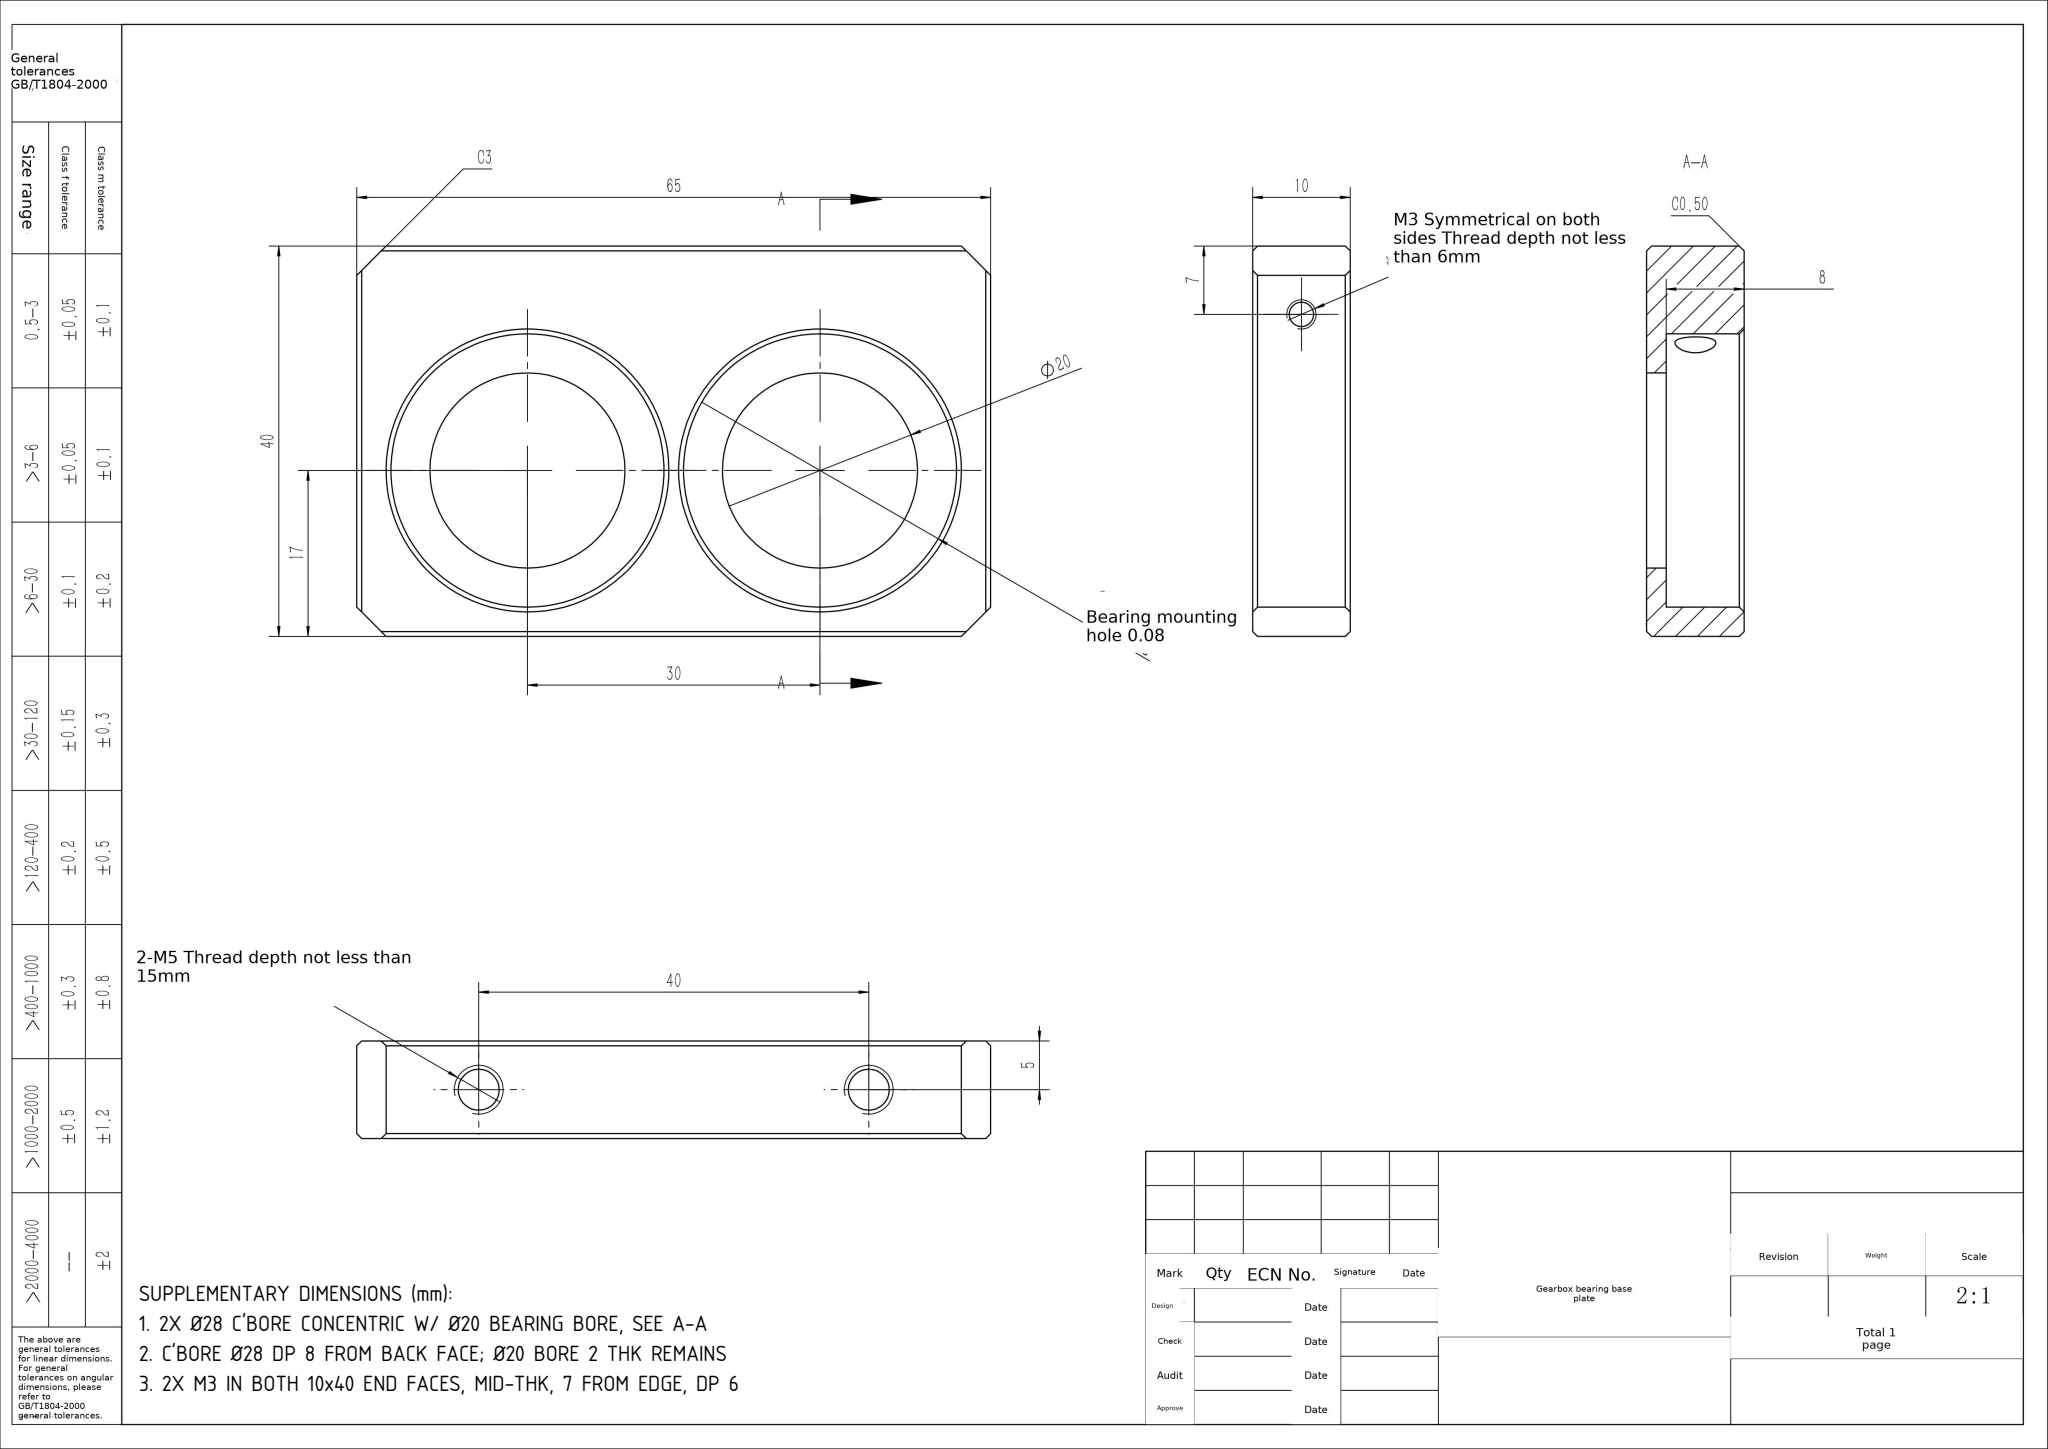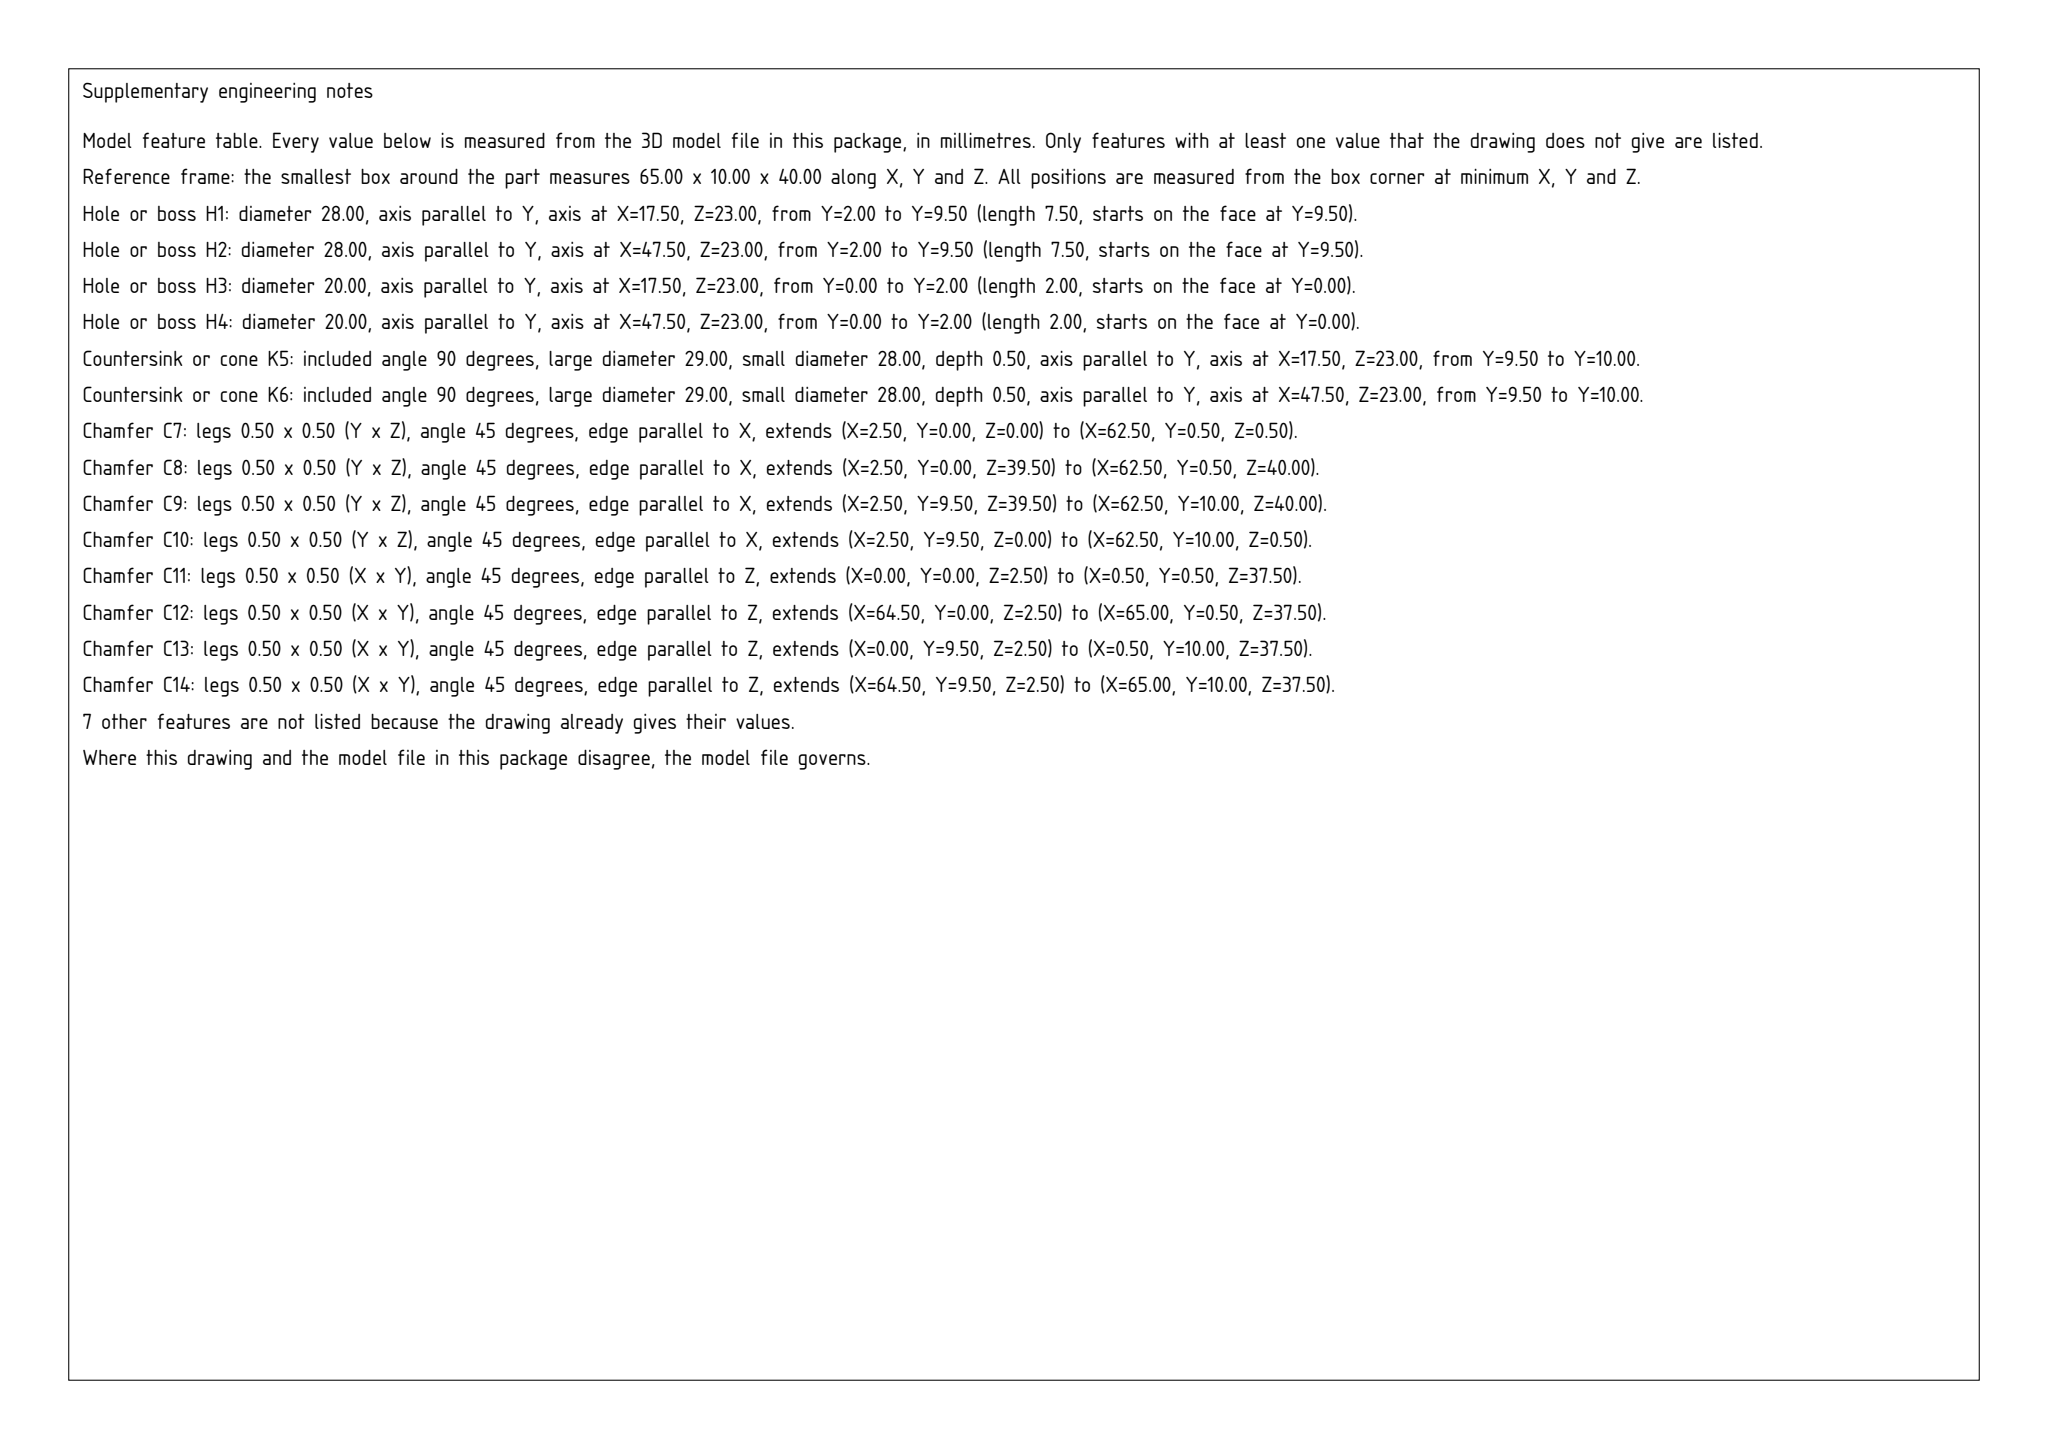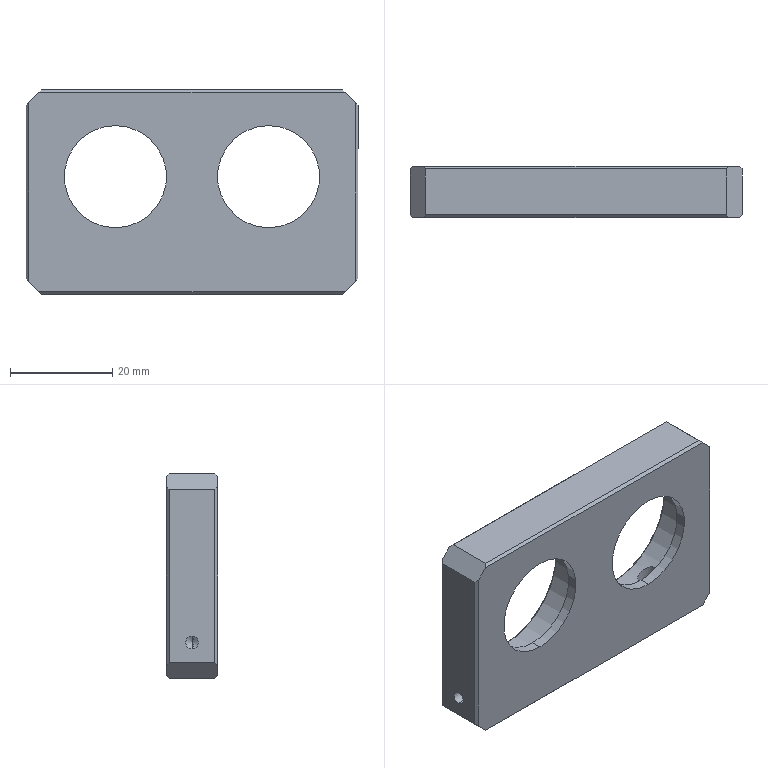Part | SolidWorks | mm | 1 solid | 44 faces | box 65 x 10 x 40 mm | volume 14290 mm3 | plane 20 | cylinder 16 | cone 8 | commonest cylinder face diameters 2.5 x4 4.2 x4 28 x4 20 x4